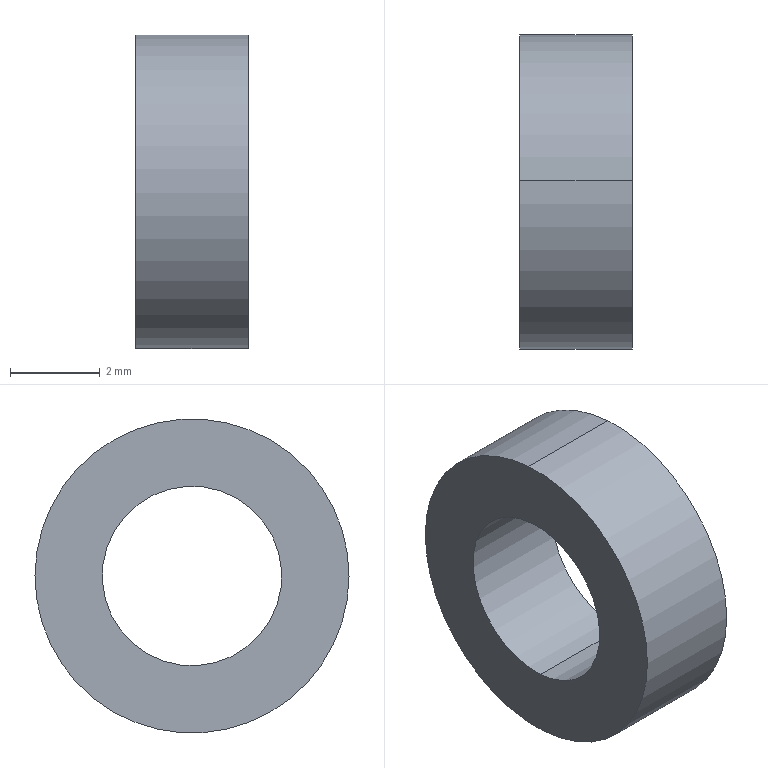Component | SolidWorks | F01AE00111-A2000-21TopEdgeAssembly-1_F01AE00111-A2000-19TopEdgeRollerAssembly-1_L-740zz--1 | 1 solid | 6 faces | box 2.5 x 7 x 7 mm | volume 65 mm3 | cylinder 4 | plane 2 | commonest cylinder face diameters 4 x2 7 x2
build123d program:
from build123d import *

# Parameters (mm, degrees)
SKETCH1_R           = 3.5
SKETCH1_R_2         = 2
BOSS_EXTRUDE1_DEPTH = 2.5


with BuildPart() as part:
    # Sketch1 → Boss-Extrude1 (new body)
    with BuildSketch(Plane(origin=(0, 0, 0), x_dir=(1, 0, 0), z_dir=(0, 1, 0))):
        with Locations(Location((0, 0, 0), (0, 0, 270))):
            Circle(SKETCH1_R)
        with Locations(Location((0, 0, 0), (0, 0, 270))):
            Circle(SKETCH1_R_2, mode=Mode.SUBTRACT)
    extrude(amount=BOSS_EXTRUDE1_DEPTH)


solid = part.part

# Placed as in the assembly
solid = solid.moved(Location((-146.352, 75.398, -381.975), (0, 0, 90)))
STEP:
#1=COLOUR_RGB('',0.7922,0.8196,0.9333);
#2=FILL_AREA_STYLE_COLOUR('',#1);
#3=FILL_AREA_STYLE('',(#2));
#4=SURFACE_STYLE_FILL_AREA(#3);
#5=SURFACE_SIDE_STYLE('',(#4));
#6=SURFACE_STYLE_USAGE(.BOTH.,#5);
#7=PRESENTATION_STYLE_ASSIGNMENT((#6));
#8=CARTESIAN_POINT('',(-5.86,2.974,-14.96));
#9=VERTEX_POINT('',#8);
#10=CARTESIAN_POINT('',(-5.86,2.963,-15.117));
#11=VERTEX_POINT('',#10);
#12=CARTESIAN_POINT('',(-5.86,2.968,-15.038));
#13=DIRECTION('',(-1.,-0.,-0.));
#14=DIRECTION('',(0.,-0.07018,-0.9975));
#15=AXIS2_PLACEMENT_3D('',#12,#13,#14);
#16=CIRCLE('',#15,0.07874);
#17=EDGE_CURVE('',#9,#11,#16,.T.);
#18=ORIENTED_EDGE('',*,*,#17,.T.);
#19=CARTESIAN_POINT('',(-5.762,2.963,-15.117));
#20=VERTEX_POINT('',#19);
#21=CARTESIAN_POINT('',(-5.86,2.963,-15.117));
#22=DIRECTION('',(1.,0.,0.));
#23=VECTOR('',#22,39.37);
#24=LINE('',#21,#23);
#25=EDGE_CURVE('',#11,#20,#24,.T.);
#26=ORIENTED_EDGE('',*,*,#25,.T.);
#27=CARTESIAN_POINT('',(-5.762,2.974,-14.96));
#28=VERTEX_POINT('',#27);
#29=CARTESIAN_POINT('',(-5.762,2.968,-15.038));
#30=DIRECTION('',(-1.,-0.,-0.));
#31=DIRECTION('',(0.,-0.07018,-0.9975));
#32=AXIS2_PLACEMENT_3D('',#29,#30,#31);
#33=CIRCLE('',#32,0.07874);
#34=EDGE_CURVE('',#28,#20,#33,.T.);
#35=ORIENTED_EDGE('',*,*,#34,.F.);
#36=CARTESIAN_POINT('',(-5.86,2.974,-14.96));
#37=DIRECTION('',(1.,0.,0.));
#38=VECTOR('',#37,39.37);
#39=LINE('',#36,#38);
#40=EDGE_CURVE('',#9,#28,#39,.T.);
#41=ORIENTED_EDGE('',*,*,#40,.F.);
#42=EDGE_LOOP('',(#18,#26,#35,#41));
#43=FACE_OUTER_BOUND('',#42,.T.);
#44=CARTESIAN_POINT('',(-5.86,2.968,-15.038));
#45=DIRECTION('',(1.,0.,0.));
#46=DIRECTION('',(0.,0.07018,0.9975));
#47=AXIS2_PLACEMENT_3D('',#44,#45,#46);
#48=CYLINDRICAL_SURFACE('',#47,0.07874);
#49=ADVANCED_FACE('',(#43),#48,.F.);
#50=CARTESIAN_POINT('',(-5.86,2.959,-15.176));
#51=VERTEX_POINT('',#50);
#52=CARTESIAN_POINT('',(-5.86,2.978,-14.901));
#53=VERTEX_POINT('',#52);
#54=CARTESIAN_POINT('',(-5.86,2.968,-15.038));
#55=DIRECTION('',(-1.,-0.,-0.));
#56=DIRECTION('',(0.,-0.07018,-0.9975));
#57=AXIS2_PLACEMENT_3D('',#54,#55,#56);
#58=CIRCLE('',#57,0.1378);
#59=EDGE_CURVE('',#51,#53,#58,.T.);
#60=ORIENTED_EDGE('',*,*,#59,.F.);
#61=CARTESIAN_POINT('',(-5.762,2.959,-15.176));
#62=VERTEX_POINT('',#61);
#63=CARTESIAN_POINT('',(-5.86,2.959,-15.176));
#64=DIRECTION('',(1.,0.,0.));
#65=VECTOR('',#64,39.37);
#66=LINE('',#63,#65);
#67=EDGE_CURVE('',#51,#62,#66,.T.);
#68=ORIENTED_EDGE('',*,*,#67,.T.);
#69=CARTESIAN_POINT('',(-5.762,2.978,-14.901));
#70=VERTEX_POINT('',#69);
#71=CARTESIAN_POINT('',(-5.762,2.968,-15.038));
#72=DIRECTION('',(-1.,-0.,-0.));
#73=DIRECTION('',(0.,-0.07018,-0.9975));
#74=AXIS2_PLACEMENT_3D('',#71,#72,#73);
#75=CIRCLE('',#74,0.1378);
#76=EDGE_CURVE('',#62,#70,#75,.T.);
#77=ORIENTED_EDGE('',*,*,#76,.T.);
#78=CARTESIAN_POINT('',(-5.86,2.978,-14.901));
#79=DIRECTION('',(1.,0.,0.));
#80=VECTOR('',#79,39.37);
#81=LINE('',#78,#80);
#82=EDGE_CURVE('',#53,#70,#81,.T.);
#83=ORIENTED_EDGE('',*,*,#82,.F.);
#84=EDGE_LOOP('',(#60,#68,#77,#83));
#85=FACE_OUTER_BOUND('',#84,.T.);
#86=CARTESIAN_POINT('',(-5.86,2.968,-15.038));
#87=DIRECTION('',(1.,0.,0.));
#88=DIRECTION('',(0.,0.07018,0.9975));
#89=AXIS2_PLACEMENT_3D('',#86,#87,#88);
#90=CYLINDRICAL_SURFACE('',#89,0.1378);
#91=ADVANCED_FACE('',(#85),#90,.T.);
#92=CARTESIAN_POINT('',(-5.86,2.968,-15.038));
#93=DIRECTION('',(-1.,-0.,-0.));
#94=DIRECTION('',(0.,-0.07018,-0.9975));
#95=AXIS2_PLACEMENT_3D('',#92,#93,#94);
#96=CIRCLE('',#95,0.1378);
#97=EDGE_CURVE('',#53,#51,#96,.T.);
#98=ORIENTED_EDGE('',*,*,#97,.T.);
#99=ORIENTED_EDGE('',*,*,#59,.T.);
#100=EDGE_LOOP('',(#98,#99));
#101=FACE_OUTER_BOUND('',#100,.T.);
#102=ORIENTED_EDGE('',*,*,#17,.F.);
#103=CARTESIAN_POINT('',(-5.86,2.968,-15.038));
#104=DIRECTION('',(-1.,-0.,-0.));
#105=DIRECTION('',(0.,-0.07018,-0.9975));
#106=AXIS2_PLACEMENT_3D('',#103,#104,#105);
#107=CIRCLE('',#106,0.07874);
#108=EDGE_CURVE('',#11,#9,#107,.T.);
#109=ORIENTED_EDGE('',*,*,#108,.F.);
#110=EDGE_LOOP('',(#102,#109));
#111=FACE_BOUND('',#110,.T.);
#112=CARTESIAN_POINT('',(-5.86,2.968,-15.038));
#113=DIRECTION('',(-1.,-0.,-0.));
#114=DIRECTION('',(0.,-0.07018,-0.9975));
#115=AXIS2_PLACEMENT_3D('',#112,#113,#114);
#116=PLANE('',#115);
#117=ADVANCED_FACE('',(#101,#111),#116,.T.);
#118=CARTESIAN_POINT('',(-5.762,2.968,-15.038));
#119=DIRECTION('',(-1.,-0.,-0.));
#120=DIRECTION('',(0.,-0.07018,-0.9975));
#121=AXIS2_PLACEMENT_3D('',#118,#119,#120);
#122=CIRCLE('',#121,0.1378);
#123=EDGE_CURVE('',#70,#62,#122,.T.);
#124=ORIENTED_EDGE('',*,*,#123,.F.);
#125=ORIENTED_EDGE('',*,*,#76,.F.);
#126=EDGE_LOOP('',(#124,#125));
#127=FACE_OUTER_BOUND('',#126,.T.);
#128=ORIENTED_EDGE('',*,*,#34,.T.);
#129=CARTESIAN_POINT('',(-5.762,2.968,-15.038));
#130=DIRECTION('',(-1.,-0.,-0.));
#131=DIRECTION('',(0.,-0.07018,-0.9975));
#132=AXIS2_PLACEMENT_3D('',#129,#130,#131);
#133=CIRCLE('',#132,0.07874);
#134=EDGE_CURVE('',#20,#28,#133,.T.);
#135=ORIENTED_EDGE('',*,*,#134,.T.);
#136=EDGE_LOOP('',(#128,#135));
#137=FACE_BOUND('',#136,.T.);
#138=CARTESIAN_POINT('',(-5.762,2.968,-15.038));
#139=DIRECTION('',(-1.,-0.,-0.));
#140=DIRECTION('',(0.,-0.07018,-0.9975));
#141=AXIS2_PLACEMENT_3D('',#138,#139,#140);
#142=PLANE('',#141);
#143=ADVANCED_FACE('',(#127,#137),#142,.F.);
#144=ORIENTED_EDGE('',*,*,#67,.F.);
#145=ORIENTED_EDGE('',*,*,#97,.F.);
#146=ORIENTED_EDGE('',*,*,#82,.T.);
#147=ORIENTED_EDGE('',*,*,#123,.T.);
#148=EDGE_LOOP('',(#144,#145,#146,#147));
#149=FACE_OUTER_BOUND('',#148,.T.);
#150=CARTESIAN_POINT('',(-5.86,2.968,-15.038));
#151=DIRECTION('',(1.,0.,0.));
#152=DIRECTION('',(0.,0.07018,0.9975));
#153=AXIS2_PLACEMENT_3D('',#150,#151,#152);
#154=CYLINDRICAL_SURFACE('',#153,0.1378);
#155=ADVANCED_FACE('',(#149),#154,.T.);
#156=ORIENTED_EDGE('',*,*,#25,.F.);
#157=ORIENTED_EDGE('',*,*,#108,.T.);
#158=ORIENTED_EDGE('',*,*,#40,.T.);
#159=ORIENTED_EDGE('',*,*,#134,.F.);
#160=EDGE_LOOP('',(#156,#157,#158,#159));
#161=FACE_OUTER_BOUND('',#160,.T.);
#162=CARTESIAN_POINT('',(-5.86,2.968,-15.038));
#163=DIRECTION('',(1.,0.,0.));
#164=DIRECTION('',(0.,0.07018,0.9975));
#165=AXIS2_PLACEMENT_3D('',#162,#163,#164);
#166=CYLINDRICAL_SURFACE('',#165,0.07874);
#167=ADVANCED_FACE('',(#161),#166,.F.);
#168=CLOSED_SHELL('',(#49,#91,#117,#143,#155,#167));
#169=MANIFOLD_SOLID_BREP('',#168);
#170=STYLED_ITEM('',(#7),#169);
#171=(LENGTH_UNIT()NAMED_UNIT(*)SI_UNIT($,.METRE.));
#172=LENGTH_MEASURE_WITH_UNIT(LENGTH_MEASURE(0.0254),#171);
#173=DIMENSIONAL_EXPONENTS(1.,0.,0.,0.,0.,0.,0.);
#174=(CONVERSION_BASED_UNIT('',#172)LENGTH_UNIT()NAMED_UNIT(#173));
#175=UNCERTAINTY_MEASURE_WITH_UNIT(LENGTH_MEASURE(0.00001),#174,'','');
#176=(NAMED_UNIT(*)PLANE_ANGLE_UNIT()SI_UNIT($,.RADIAN.));
#177=(NAMED_UNIT(*)SI_UNIT($,.STERADIAN.)SOLID_ANGLE_UNIT());
#178=(GEOMETRIC_REPRESENTATION_CONTEXT(3)GLOBAL_UNCERTAINTY_ASSIGNED_CONTEXT((#175))GLOBAL_UNIT_ASSIGNED_CONTEXT((#174,#176,#177))REPRESENTATION_CONTEXT('',''));
#179=MECHANICAL_DESIGN_GEOMETRIC_PRESENTATION_REPRESENTATION('',(#170),#178);
#180=CARTESIAN_POINT('',(0.,0.,0.));
#181=DIRECTION('',(0.,0.,1.));
#182=DIRECTION('',(1.,0.,0.));
#183=AXIS2_PLACEMENT_3D('',#180,#181,#182);
#184=(LENGTH_UNIT()NAMED_UNIT(*)SI_UNIT($,.METRE.));
#185=LENGTH_MEASURE_WITH_UNIT(LENGTH_MEASURE(0.0254),#184);
#186=DIMENSIONAL_EXPONENTS(1.,0.,0.,0.,0.,0.,0.);
#187=(CONVERSION_BASED_UNIT('',#185)LENGTH_UNIT()NAMED_UNIT(#186));
#188=UNCERTAINTY_MEASURE_WITH_UNIT(LENGTH_MEASURE(0.00001),#187,'','');
#189=(NAMED_UNIT(*)PLANE_ANGLE_UNIT()SI_UNIT($,.RADIAN.));
#190=(NAMED_UNIT(*)SI_UNIT($,.STERADIAN.)SOLID_ANGLE_UNIT());
#191=(GEOMETRIC_REPRESENTATION_CONTEXT(3)GLOBAL_UNCERTAINTY_ASSIGNED_CONTEXT((#188))GLOBAL_UNIT_ASSIGNED_CONTEXT((#187,#189,#190))REPRESENTATION_CONTEXT('',''));
#192=ADVANCED_BREP_SHAPE_REPRESENTATION('',(#169,#183),#191);
#193=PRESENTATION_LAYER_ASSIGNMENT('','',(#170));